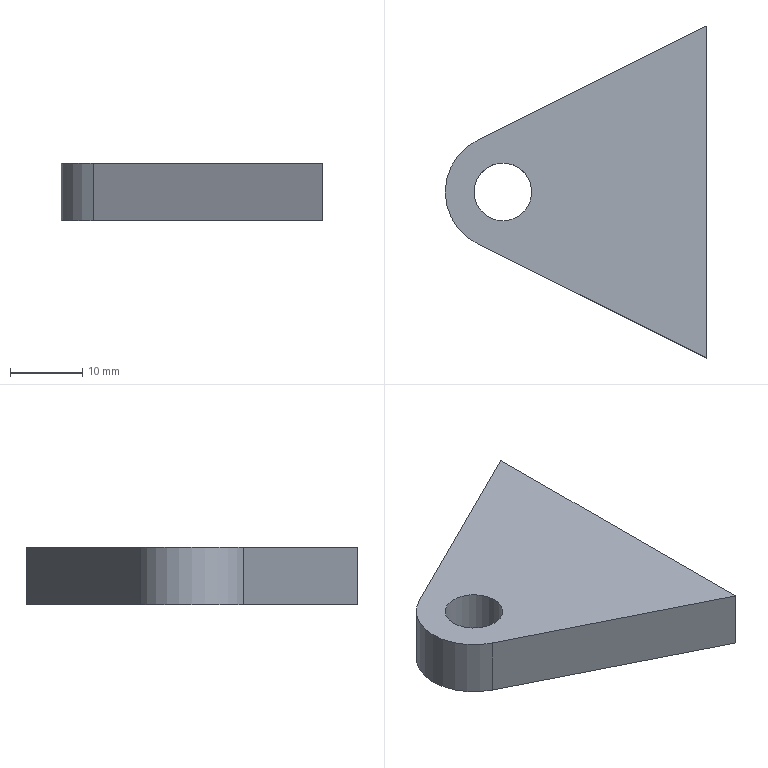Component | NX | FIXED_BASE_2 | 1 solid | 7 faces | box 36.29 x 46.04 x 8 mm | volume 7654 mm3 | plane 5 | cylinder 2 | commonest cylinder face diameters 16 x1 8 x1
STEP:
#1=CARTESIAN_POINT('',(0.,0.,0.));
#2=DIRECTION('',(0.,0.,1.));
#3=DIRECTION('',(1.,0.,0.));
#4=AXIS2_PLACEMENT_3D('',#1,#2,#3);
#5=CARTESIAN_POINT('',(50.435,7.162,-12.));
#6=VERTEX_POINT('',#5);
#7=CARTESIAN_POINT('',(50.435,-7.162,-12.));
#8=VERTEX_POINT('',#7);
#9=CARTESIAN_POINT('',(54.,0.,-12.));
#10=DIRECTION('',(0.,0.,1.));
#11=DIRECTION('',(1.,0.,0.));
#12=AXIS2_PLACEMENT_3D('',#9,#10,#11);
#13=CIRCLE('',#12,8.);
#14=CARTESIAN_POINT('',(54.,0.,-4.));
#15=DIRECTION('',(0.,0.,-1.));
#16=DIRECTION('',(-1.,0.,0.));
#17=AXIS2_PLACEMENT_3D('',#14,#15,#16);
#18=CYLINDRICAL_SURFACE('',#17,8.);
#19=CARTESIAN_POINT('',(3.142,8.));
#20=DIRECTION('',(-1.,0.));
#21=VECTOR('',#20,1.);
#22=LINE('',#19,#21);
#23=(GEOMETRIC_REPRESENTATION_CONTEXT(2)PARAMETRIC_REPRESENTATION_CONTEXT()REPRESENTATION_CONTEXT('',''));
#24=DEFINITIONAL_REPRESENTATION('',(#22),#23);
#25=PCURVE('',#18,#24);
#26=CARTESIAN_POINT('',(54.,0.,-12.));
#27=DIRECTION('',(0.,0.,1.));
#28=DIRECTION('',(1.,0.,0.));
#29=AXIS2_PLACEMENT_3D('',#26,#27,#28);
#30=PLANE('',#29);
#31=CARTESIAN_POINT('',(0.,0.));
#32=DIRECTION('',(1.,0.));
#33=AXIS2_PLACEMENT_2D('',#31,#32);
#34=CIRCLE('',#33,8.);
#35=(GEOMETRIC_REPRESENTATION_CONTEXT(2)PARAMETRIC_REPRESENTATION_CONTEXT()REPRESENTATION_CONTEXT('',''));
#36=DEFINITIONAL_REPRESENTATION('',(#34),#35);
#37=PCURVE('',#30,#36);
#38=SURFACE_CURVE('',#13,(#25,#37),.PCURVE_S1.);
#39=EDGE_CURVE('',#6,#8,#38,.T.);
#40=ORIENTED_EDGE('',*,*,#39,.T.);
#41=CARTESIAN_POINT('',(50.435,-7.162,-4.));
#42=VERTEX_POINT('',#41);
#43=CARTESIAN_POINT('',(50.435,-7.162,-4.));
#44=DIRECTION('',(0.,0.,-1.));
#45=VECTOR('',#44,1.);
#46=LINE('',#43,#45);
#47=CARTESIAN_POINT('',(-1.109,0.));
#48=DIRECTION('',(0.,1.));
#49=VECTOR('',#48,1.);
#50=LINE('',#47,#49);
#51=(GEOMETRIC_REPRESENTATION_CONTEXT(2)PARAMETRIC_REPRESENTATION_CONTEXT()REPRESENTATION_CONTEXT('',''));
#52=DEFINITIONAL_REPRESENTATION('',(#50),#51);
#53=PCURVE('',#18,#52);
#54=CARTESIAN_POINT('',(50.435,-7.162,-4.));
#55=DIRECTION('',(0.4456,0.8952,0.));
#56=DIRECTION('',(-0.8952,0.4456,0.));
#57=AXIS2_PLACEMENT_3D('',#54,#55,#56);
#58=PLANE('',#57);
#59=CARTESIAN_POINT('',(0.,0.));
#60=DIRECTION('',(0.,-1.));
#61=VECTOR('',#60,1.);
#62=LINE('',#59,#61);
#63=(GEOMETRIC_REPRESENTATION_CONTEXT(2)PARAMETRIC_REPRESENTATION_CONTEXT()REPRESENTATION_CONTEXT('',''));
#64=DEFINITIONAL_REPRESENTATION('',(#62),#63);
#65=PCURVE('',#58,#64);
#66=SURFACE_CURVE('',#46,(#53,#65),.PCURVE_S1.);
#67=EDGE_CURVE('',#42,#8,#66,.T.);
#68=ORIENTED_EDGE('',*,*,#67,.F.);
#69=CARTESIAN_POINT('',(50.435,7.162,-4.));
#70=VERTEX_POINT('',#69);
#71=CARTESIAN_POINT('',(54.,0.,-4.));
#72=DIRECTION('',(0.,0.,1.));
#73=DIRECTION('',(1.,0.,0.));
#74=AXIS2_PLACEMENT_3D('',#71,#72,#73);
#75=CIRCLE('',#74,8.);
#76=CARTESIAN_POINT('',(3.142,0.));
#77=DIRECTION('',(-1.,0.));
#78=VECTOR('',#77,1.);
#79=LINE('',#76,#78);
#80=(GEOMETRIC_REPRESENTATION_CONTEXT(2)PARAMETRIC_REPRESENTATION_CONTEXT()REPRESENTATION_CONTEXT('',''));
#81=DEFINITIONAL_REPRESENTATION('',(#79),#80);
#82=PCURVE('',#18,#81);
#83=CARTESIAN_POINT('',(54.,0.,-4.));
#84=DIRECTION('',(0.,0.,1.));
#85=DIRECTION('',(1.,0.,0.));
#86=AXIS2_PLACEMENT_3D('',#83,#84,#85);
#87=PLANE('',#86);
#88=CARTESIAN_POINT('',(0.,0.));
#89=DIRECTION('',(1.,0.));
#90=AXIS2_PLACEMENT_2D('',#88,#89);
#91=CIRCLE('',#90,8.);
#92=(GEOMETRIC_REPRESENTATION_CONTEXT(2)PARAMETRIC_REPRESENTATION_CONTEXT()REPRESENTATION_CONTEXT('',''));
#93=DEFINITIONAL_REPRESENTATION('',(#91),#92);
#94=PCURVE('',#87,#93);
#95=SURFACE_CURVE('',#75,(#82,#94),.PCURVE_S1.);
#96=EDGE_CURVE('',#70,#42,#95,.T.);
#97=ORIENTED_EDGE('',*,*,#96,.F.);
#98=CARTESIAN_POINT('',(50.435,7.162,-4.));
#99=DIRECTION('',(0.,0.,-1.));
#100=VECTOR('',#99,1.);
#101=LINE('',#98,#100);
#102=CARTESIAN_POINT('',(1.109,0.));
#103=DIRECTION('',(0.,1.));
#104=VECTOR('',#103,1.);
#105=LINE('',#102,#104);
#106=(GEOMETRIC_REPRESENTATION_CONTEXT(2)PARAMETRIC_REPRESENTATION_CONTEXT()REPRESENTATION_CONTEXT('',''));
#107=DEFINITIONAL_REPRESENTATION('',(#105),#106);
#108=PCURVE('',#18,#107);
#109=CARTESIAN_POINT('',(82.294,23.02,-4.));
#110=DIRECTION('',(0.4456,-0.8952,0.));
#111=DIRECTION('',(0.8952,0.4456,0.));
#112=AXIS2_PLACEMENT_3D('',#109,#110,#111);
#113=PLANE('',#112);
#114=CARTESIAN_POINT('',(-35.587,0.));
#115=DIRECTION('',(0.,-1.));
#116=VECTOR('',#115,1.);
#117=LINE('',#114,#116);
#118=(GEOMETRIC_REPRESENTATION_CONTEXT(2)PARAMETRIC_REPRESENTATION_CONTEXT()REPRESENTATION_CONTEXT('',''));
#119=DEFINITIONAL_REPRESENTATION('',(#117),#118);
#120=PCURVE('',#113,#119);
#121=SURFACE_CURVE('',#101,(#108,#120),.PCURVE_S1.);
#122=EDGE_CURVE('',#70,#6,#121,.T.);
#123=ORIENTED_EDGE('',*,*,#122,.T.);
#124=EDGE_LOOP('',(#40,#68,#97,#123));
#125=FACE_BOUND('',#124,.T.);
#126=ADVANCED_FACE('',(#125),#18,.T.);
#127=CARTESIAN_POINT('',(82.294,-23.02,-12.));
#128=VERTEX_POINT('',#127);
#129=CARTESIAN_POINT('',(50.435,-7.162,-12.));
#130=DIRECTION('',(0.8952,-0.4456,0.));
#131=VECTOR('',#130,1.);
#132=LINE('',#129,#131);
#133=CARTESIAN_POINT('',(0.,-8.));
#134=DIRECTION('',(-1.,0.));
#135=VECTOR('',#134,1.);
#136=LINE('',#133,#135);
#137=(GEOMETRIC_REPRESENTATION_CONTEXT(2)PARAMETRIC_REPRESENTATION_CONTEXT()REPRESENTATION_CONTEXT('',''));
#138=DEFINITIONAL_REPRESENTATION('',(#136),#137);
#139=PCURVE('',#58,#138);
#140=CARTESIAN_POINT('',(-3.565,-7.162));
#141=DIRECTION('',(0.8952,-0.4456));
#142=VECTOR('',#141,1.);
#143=LINE('',#140,#142);
#144=(GEOMETRIC_REPRESENTATION_CONTEXT(2)PARAMETRIC_REPRESENTATION_CONTEXT()REPRESENTATION_CONTEXT('',''));
#145=DEFINITIONAL_REPRESENTATION('',(#143),#144);
#146=PCURVE('',#30,#145);
#147=SURFACE_CURVE('',#132,(#139,#146),.PCURVE_S1.);
#148=EDGE_CURVE('',#8,#128,#147,.T.);
#149=ORIENTED_EDGE('',*,*,#148,.T.);
#150=CARTESIAN_POINT('',(82.294,-23.02,-4.));
#151=VERTEX_POINT('',#150);
#152=CARTESIAN_POINT('',(82.294,-23.02,-4.));
#153=DIRECTION('',(0.,0.,-1.));
#154=VECTOR('',#153,1.);
#155=LINE('',#152,#154);
#156=CARTESIAN_POINT('',(-35.587,0.));
#157=DIRECTION('',(0.,-1.));
#158=VECTOR('',#157,1.);
#159=LINE('',#156,#158);
#160=(GEOMETRIC_REPRESENTATION_CONTEXT(2)PARAMETRIC_REPRESENTATION_CONTEXT()REPRESENTATION_CONTEXT('',''));
#161=DEFINITIONAL_REPRESENTATION('',(#159),#160);
#162=PCURVE('',#58,#161);
#163=CARTESIAN_POINT('',(82.294,-23.02,-4.));
#164=DIRECTION('',(-1.,0.,0.));
#165=DIRECTION('',(-0.,-1.,0.));
#166=AXIS2_PLACEMENT_3D('',#163,#164,#165);
#167=PLANE('',#166);
#168=CARTESIAN_POINT('',(0.,0.));
#169=DIRECTION('',(0.,-1.));
#170=VECTOR('',#169,1.);
#171=LINE('',#168,#170);
#172=(GEOMETRIC_REPRESENTATION_CONTEXT(2)PARAMETRIC_REPRESENTATION_CONTEXT()REPRESENTATION_CONTEXT('',''));
#173=DEFINITIONAL_REPRESENTATION('',(#171),#172);
#174=PCURVE('',#167,#173);
#175=SURFACE_CURVE('',#155,(#162,#174),.PCURVE_S1.);
#176=EDGE_CURVE('',#151,#128,#175,.T.);
#177=ORIENTED_EDGE('',*,*,#176,.F.);
#178=CARTESIAN_POINT('',(50.435,-7.162,-4.));
#179=DIRECTION('',(0.8952,-0.4456,0.));
#180=VECTOR('',#179,1.);
#181=LINE('',#178,#180);
#182=CARTESIAN_POINT('',(0.,0.));
#183=DIRECTION('',(-1.,0.));
#184=VECTOR('',#183,1.);
#185=LINE('',#182,#184);
#186=(GEOMETRIC_REPRESENTATION_CONTEXT(2)PARAMETRIC_REPRESENTATION_CONTEXT()REPRESENTATION_CONTEXT('',''));
#187=DEFINITIONAL_REPRESENTATION('',(#185),#186);
#188=PCURVE('',#58,#187);
#189=CARTESIAN_POINT('',(-3.565,-7.162));
#190=DIRECTION('',(0.8952,-0.4456));
#191=VECTOR('',#190,1.);
#192=LINE('',#189,#191);
#193=(GEOMETRIC_REPRESENTATION_CONTEXT(2)PARAMETRIC_REPRESENTATION_CONTEXT()REPRESENTATION_CONTEXT('',''));
#194=DEFINITIONAL_REPRESENTATION('',(#192),#193);
#195=PCURVE('',#87,#194);
#196=SURFACE_CURVE('',#181,(#188,#195),.PCURVE_S1.);
#197=EDGE_CURVE('',#42,#151,#196,.T.);
#198=ORIENTED_EDGE('',*,*,#197,.F.);
#199=ORIENTED_EDGE('',*,*,#67,.T.);
#200=EDGE_LOOP('',(#149,#177,#198,#199));
#201=FACE_BOUND('',#200,.T.);
#202=ADVANCED_FACE('',(#201),#58,.F.);
#203=CARTESIAN_POINT('',(82.294,23.02,-12.));
#204=VERTEX_POINT('',#203);
#205=CARTESIAN_POINT('',(82.294,-23.02,-12.));
#206=DIRECTION('',(0.,1.,0.));
#207=VECTOR('',#206,1.);
#208=LINE('',#205,#207);
#209=CARTESIAN_POINT('',(0.,-8.));
#210=DIRECTION('',(-1.,0.));
#211=VECTOR('',#210,1.);
#212=LINE('',#209,#211);
#213=(GEOMETRIC_REPRESENTATION_CONTEXT(2)PARAMETRIC_REPRESENTATION_CONTEXT()REPRESENTATION_CONTEXT('',''));
#214=DEFINITIONAL_REPRESENTATION('',(#212),#213);
#215=PCURVE('',#167,#214);
#216=CARTESIAN_POINT('',(28.294,-23.02));
#217=DIRECTION('',(0.,1.));
#218=VECTOR('',#217,1.);
#219=LINE('',#216,#218);
#220=(GEOMETRIC_REPRESENTATION_CONTEXT(2)PARAMETRIC_REPRESENTATION_CONTEXT()REPRESENTATION_CONTEXT('',''));
#221=DEFINITIONAL_REPRESENTATION('',(#219),#220);
#222=PCURVE('',#30,#221);
#223=SURFACE_CURVE('',#208,(#215,#222),.PCURVE_S1.);
#224=EDGE_CURVE('',#128,#204,#223,.T.);
#225=ORIENTED_EDGE('',*,*,#224,.T.);
#226=CARTESIAN_POINT('',(82.294,23.02,-4.));
#227=VERTEX_POINT('',#226);
#228=CARTESIAN_POINT('',(82.294,23.02,-4.));
#229=DIRECTION('',(0.,0.,-1.));
#230=VECTOR('',#229,1.);
#231=LINE('',#228,#230);
#232=CARTESIAN_POINT('',(-46.039,0.));
#233=DIRECTION('',(0.,-1.));
#234=VECTOR('',#233,1.);
#235=LINE('',#232,#234);
#236=(GEOMETRIC_REPRESENTATION_CONTEXT(2)PARAMETRIC_REPRESENTATION_CONTEXT()REPRESENTATION_CONTEXT('',''));
#237=DEFINITIONAL_REPRESENTATION('',(#235),#236);
#238=PCURVE('',#167,#237);
#239=CARTESIAN_POINT('',(0.,0.));
#240=DIRECTION('',(0.,-1.));
#241=VECTOR('',#240,1.);
#242=LINE('',#239,#241);
#243=(GEOMETRIC_REPRESENTATION_CONTEXT(2)PARAMETRIC_REPRESENTATION_CONTEXT()REPRESENTATION_CONTEXT('',''));
#244=DEFINITIONAL_REPRESENTATION('',(#242),#243);
#245=PCURVE('',#113,#244);
#246=SURFACE_CURVE('',#231,(#238,#245),.PCURVE_S1.);
#247=EDGE_CURVE('',#227,#204,#246,.T.);
#248=ORIENTED_EDGE('',*,*,#247,.F.);
#249=CARTESIAN_POINT('',(82.294,-23.02,-4.));
#250=DIRECTION('',(0.,1.,0.));
#251=VECTOR('',#250,1.);
#252=LINE('',#249,#251);
#253=CARTESIAN_POINT('',(0.,0.));
#254=DIRECTION('',(-1.,0.));
#255=VECTOR('',#254,1.);
#256=LINE('',#253,#255);
#257=(GEOMETRIC_REPRESENTATION_CONTEXT(2)PARAMETRIC_REPRESENTATION_CONTEXT()REPRESENTATION_CONTEXT('',''));
#258=DEFINITIONAL_REPRESENTATION('',(#256),#257);
#259=PCURVE('',#167,#258);
#260=CARTESIAN_POINT('',(28.294,-23.02));
#261=DIRECTION('',(0.,1.));
#262=VECTOR('',#261,1.);
#263=LINE('',#260,#262);
#264=(GEOMETRIC_REPRESENTATION_CONTEXT(2)PARAMETRIC_REPRESENTATION_CONTEXT()REPRESENTATION_CONTEXT('',''));
#265=DEFINITIONAL_REPRESENTATION('',(#263),#264);
#266=PCURVE('',#87,#265);
#267=SURFACE_CURVE('',#252,(#259,#266),.PCURVE_S1.);
#268=EDGE_CURVE('',#151,#227,#267,.T.);
#269=ORIENTED_EDGE('',*,*,#268,.F.);
#270=ORIENTED_EDGE('',*,*,#176,.T.);
#271=EDGE_LOOP('',(#225,#248,#269,#270));
#272=FACE_BOUND('',#271,.T.);
#273=ADVANCED_FACE('',(#272),#167,.F.);
#274=CARTESIAN_POINT('',(82.294,23.02,-12.));
#275=DIRECTION('',(-0.8952,-0.4456,0.));
#276=VECTOR('',#275,1.);
#277=LINE('',#274,#276);
#278=CARTESIAN_POINT('',(0.,-8.));
#279=DIRECTION('',(-1.,0.));
#280=VECTOR('',#279,1.);
#281=LINE('',#278,#280);
#282=(GEOMETRIC_REPRESENTATION_CONTEXT(2)PARAMETRIC_REPRESENTATION_CONTEXT()REPRESENTATION_CONTEXT('',''));
#283=DEFINITIONAL_REPRESENTATION('',(#281),#282);
#284=PCURVE('',#113,#283);
#285=CARTESIAN_POINT('',(28.294,23.02));
#286=DIRECTION('',(-0.8952,-0.4456));
#287=VECTOR('',#286,1.);
#288=LINE('',#285,#287);
#289=(GEOMETRIC_REPRESENTATION_CONTEXT(2)PARAMETRIC_REPRESENTATION_CONTEXT()REPRESENTATION_CONTEXT('',''));
#290=DEFINITIONAL_REPRESENTATION('',(#288),#289);
#291=PCURVE('',#30,#290);
#292=SURFACE_CURVE('',#277,(#284,#291),.PCURVE_S1.);
#293=EDGE_CURVE('',#204,#6,#292,.T.);
#294=ORIENTED_EDGE('',*,*,#293,.T.);
#295=ORIENTED_EDGE('',*,*,#122,.F.);
#296=CARTESIAN_POINT('',(82.294,23.02,-4.));
#297=DIRECTION('',(-0.8952,-0.4456,0.));
#298=VECTOR('',#297,1.);
#299=LINE('',#296,#298);
#300=CARTESIAN_POINT('',(0.,0.));
#301=DIRECTION('',(-1.,0.));
#302=VECTOR('',#301,1.);
#303=LINE('',#300,#302);
#304=(GEOMETRIC_REPRESENTATION_CONTEXT(2)PARAMETRIC_REPRESENTATION_CONTEXT()REPRESENTATION_CONTEXT('',''));
#305=DEFINITIONAL_REPRESENTATION('',(#303),#304);
#306=PCURVE('',#113,#305);
#307=CARTESIAN_POINT('',(28.294,23.02));
#308=DIRECTION('',(-0.8952,-0.4456));
#309=VECTOR('',#308,1.);
#310=LINE('',#307,#309);
#311=(GEOMETRIC_REPRESENTATION_CONTEXT(2)PARAMETRIC_REPRESENTATION_CONTEXT()REPRESENTATION_CONTEXT('',''));
#312=DEFINITIONAL_REPRESENTATION('',(#310),#311);
#313=PCURVE('',#87,#312);
#314=SURFACE_CURVE('',#299,(#306,#313),.PCURVE_S1.);
#315=EDGE_CURVE('',#227,#70,#314,.T.);
#316=ORIENTED_EDGE('',*,*,#315,.F.);
#317=ORIENTED_EDGE('',*,*,#247,.T.);
#318=EDGE_LOOP('',(#294,#295,#316,#317));
#319=FACE_BOUND('',#318,.T.);
#320=ADVANCED_FACE('',(#319),#113,.F.);
#321=CARTESIAN_POINT('',(58.,0.,-4.));
#322=VERTEX_POINT('',#321);
#323=CARTESIAN_POINT('',(54.,0.,-4.));
#324=DIRECTION('',(0.,0.,1.));
#325=DIRECTION('',(1.,0.,0.));
#326=AXIS2_PLACEMENT_3D('',#323,#324,#325);
#327=CIRCLE('',#326,4.);
#328=CARTESIAN_POINT('',(54.,0.,-4.));
#329=DIRECTION('',(0.,0.,-1.));
#330=DIRECTION('',(-1.,0.,0.));
#331=AXIS2_PLACEMENT_3D('',#328,#329,#330);
#332=CYLINDRICAL_SURFACE('',#331,4.);
#333=CARTESIAN_POINT('',(9.425,0.));
#334=DIRECTION('',(-1.,0.));
#335=VECTOR('',#334,1.);
#336=LINE('',#333,#335);
#337=(GEOMETRIC_REPRESENTATION_CONTEXT(2)PARAMETRIC_REPRESENTATION_CONTEXT()REPRESENTATION_CONTEXT('',''));
#338=DEFINITIONAL_REPRESENTATION('',(#336),#337);
#339=PCURVE('',#332,#338);
#340=CARTESIAN_POINT('',(0.,0.));
#341=DIRECTION('',(1.,0.));
#342=AXIS2_PLACEMENT_2D('',#340,#341);
#343=CIRCLE('',#342,4.);
#344=(GEOMETRIC_REPRESENTATION_CONTEXT(2)PARAMETRIC_REPRESENTATION_CONTEXT()REPRESENTATION_CONTEXT('',''));
#345=DEFINITIONAL_REPRESENTATION('',(#343),#344);
#346=PCURVE('',#87,#345);
#347=SURFACE_CURVE('',#327,(#339,#346),.PCURVE_S1.);
#348=EDGE_CURVE('',#322,#322,#347,.T.);
#349=ORIENTED_EDGE('',*,*,#348,.F.);
#350=CARTESIAN_POINT('',(58.,0.,-12.));
#351=VERTEX_POINT('',#350);
#352=CARTESIAN_POINT('',(58.,0.,-4.));
#353=CARTESIAN_POINT('',(58.,0.,-12.));
#354=B_SPLINE_CURVE_WITH_KNOTS('',1,(#352,#353),.UNSPECIFIED.,.F.,.F.,(2,2),(0.,8.),.PIECEWISE_BEZIER_KNOTS.);
#355=CARTESIAN_POINT('',(9.425,0.));
#356=DIRECTION('',(0.,1.));
#357=VECTOR('',#356,1.);
#358=LINE('',#355,#357);
#359=(GEOMETRIC_REPRESENTATION_CONTEXT(2)PARAMETRIC_REPRESENTATION_CONTEXT()REPRESENTATION_CONTEXT('',''));
#360=DEFINITIONAL_REPRESENTATION('',(#358),#359);
#361=PCURVE('',#332,#360);
#362=CARTESIAN_POINT('',(3.142,0.));
#363=DIRECTION('',(0.,1.));
#364=VECTOR('',#363,1.);
#365=LINE('',#362,#364);
#366=(GEOMETRIC_REPRESENTATION_CONTEXT(2)PARAMETRIC_REPRESENTATION_CONTEXT()REPRESENTATION_CONTEXT('',''));
#367=DEFINITIONAL_REPRESENTATION('',(#365),#366);
#368=PCURVE('',#332,#367);
#369=SEAM_CURVE('',#354,(#361,#368),.PCURVE_S1.);
#370=EDGE_CURVE('',#322,#351,#369,.T.);
#371=ORIENTED_EDGE('',*,*,#370,.T.);
#372=CARTESIAN_POINT('',(54.,0.,-12.));
#373=DIRECTION('',(0.,0.,1.));
#374=DIRECTION('',(1.,0.,0.));
#375=AXIS2_PLACEMENT_3D('',#372,#373,#374);
#376=CIRCLE('',#375,4.);
#377=CARTESIAN_POINT('',(9.425,8.));
#378=DIRECTION('',(-1.,0.));
#379=VECTOR('',#378,1.);
#380=LINE('',#377,#379);
#381=(GEOMETRIC_REPRESENTATION_CONTEXT(2)PARAMETRIC_REPRESENTATION_CONTEXT()REPRESENTATION_CONTEXT('',''));
#382=DEFINITIONAL_REPRESENTATION('',(#380),#381);
#383=PCURVE('',#332,#382);
#384=CARTESIAN_POINT('',(0.,0.));
#385=DIRECTION('',(1.,0.));
#386=AXIS2_PLACEMENT_2D('',#384,#385);
#387=CIRCLE('',#386,4.);
#388=(GEOMETRIC_REPRESENTATION_CONTEXT(2)PARAMETRIC_REPRESENTATION_CONTEXT()REPRESENTATION_CONTEXT('',''));
#389=DEFINITIONAL_REPRESENTATION('',(#387),#388);
#390=PCURVE('',#30,#389);
#391=SURFACE_CURVE('',#376,(#383,#390),.PCURVE_S1.);
#392=EDGE_CURVE('',#351,#351,#391,.T.);
#393=ORIENTED_EDGE('',*,*,#392,.T.);
#394=ORIENTED_EDGE('',*,*,#370,.F.);
#395=EDGE_LOOP('',(#349,#371,#393,#394));
#396=FACE_BOUND('',#395,.F.);
#397=ADVANCED_FACE('',(#396),#332,.F.);
#398=ORIENTED_EDGE('',*,*,#96,.T.);
#399=ORIENTED_EDGE('',*,*,#197,.T.);
#400=ORIENTED_EDGE('',*,*,#268,.T.);
#401=ORIENTED_EDGE('',*,*,#315,.T.);
#402=EDGE_LOOP('',(#398,#399,#400,#401));
#403=FACE_BOUND('',#402,.T.);
#404=ORIENTED_EDGE('',*,*,#348,.F.);
#405=EDGE_LOOP('',(#404));
#406=FACE_BOUND('',#405,.T.);
#407=ADVANCED_FACE('',(#403,#406),#87,.T.);
#408=ORIENTED_EDGE('',*,*,#39,.F.);
#409=ORIENTED_EDGE('',*,*,#293,.F.);
#410=ORIENTED_EDGE('',*,*,#224,.F.);
#411=ORIENTED_EDGE('',*,*,#148,.F.);
#412=EDGE_LOOP('',(#408,#409,#410,#411));
#413=FACE_BOUND('',#412,.T.);
#414=ORIENTED_EDGE('',*,*,#392,.T.);
#415=EDGE_LOOP('',(#414));
#416=FACE_BOUND('',#415,.T.);
#417=ADVANCED_FACE('',(#413,#416),#30,.F.);
#418=CLOSED_SHELL('',(#126,#202,#273,#320,#397,#407,#417));
#419=MANIFOLD_SOLID_BREP('',#418);
#420=(LENGTH_UNIT()NAMED_UNIT(*)SI_UNIT(.MILLI.,.METRE.));
#421=UNCERTAINTY_MEASURE_WITH_UNIT(LENGTH_MEASURE(0.000002),#420,'','');
#422=(NAMED_UNIT(*)PLANE_ANGLE_UNIT()SI_UNIT($,.RADIAN.));
#423=(NAMED_UNIT(*)SI_UNIT($,.STERADIAN.)SOLID_ANGLE_UNIT());
#424=(GEOMETRIC_REPRESENTATION_CONTEXT(3)GLOBAL_UNCERTAINTY_ASSIGNED_CONTEXT((#421))GLOBAL_UNIT_ASSIGNED_CONTEXT((#420,#422,#423))REPRESENTATION_CONTEXT('',''));
#425=ADVANCED_BREP_SHAPE_REPRESENTATION('',(#4,#419),#424);